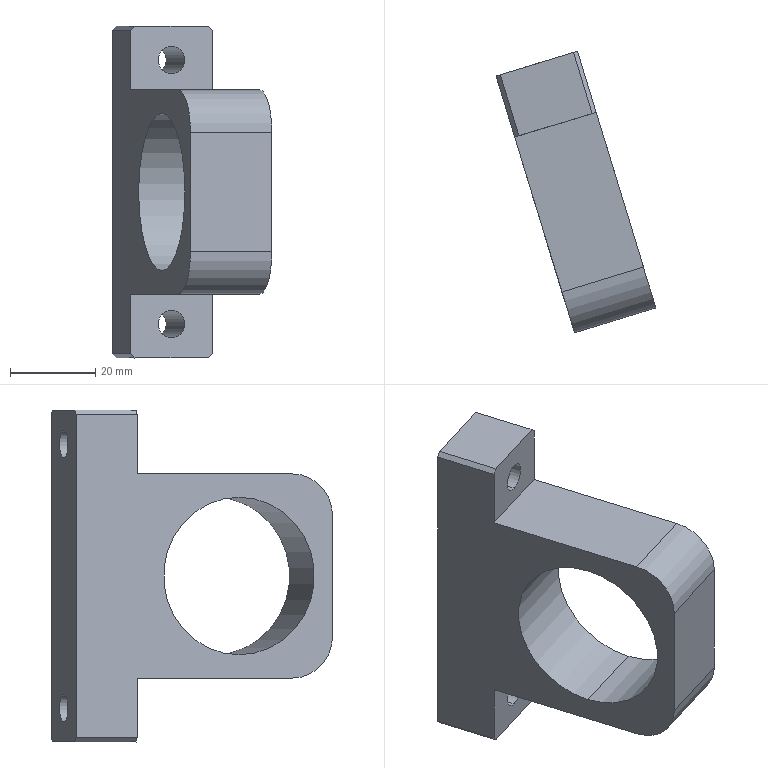Component | SolidWorks | V1ZHXTRotatingAxisMountingBaseSB1-1 | 1 solid | 22 faces | box 37.51 x 66.09 x 78 mm | volume 46092 mm3 | plane 14 | cylinder 8 | commonest cylinder face diameters 6.5 x4 37 x2 20 x2
build123d program:
from build123d import *

# Parameters (mm, degrees)
SKETCH1_W           = 20
SKETCH1_H           = 78
BOSS_EXTRUDE1_DEPTH = 63
SKETCH2_R           = 18.5
CUT_EXTRUDE1_DEPTH  = 77.746
SKETCH3_W           = 20
SKETCH3_H           = 15
CUT_EXTRUDE2_DEPTH  = 48
FILLET1_R           = 10
CHAMFER1_SIZE       = 1
SKETCH5_R           = 3.25
CUT_EXTRUDE3_DEPTH  = 66


with BuildPart() as part:
    # Sketch1 → Boss-Extrude1 (new body)
    with BuildSketch(Plane(origin=(0, 0, 0), x_dir=(1, 0, 0), z_dir=(0, 1, 0))):
        with Locations((10, 0)):
            Rectangle(SKETCH1_W, SKETCH1_H)
    extrude(amount=BOSS_EXTRUDE1_DEPTH)

    # Sketch2 → Cut-Extrude1 (cut, through all)
    with BuildSketch(Plane.ZY):
        with Locations((0, 40)):
            Circle(SKETCH2_R)
    extrude(amount=-CUT_EXTRUDE1_DEPTH, mode=Mode.SUBTRACT)

    # Sketch3 → Cut-Extrude2 (cut)
    with BuildSketch(Plane(origin=(0, 63, 0), x_dir=(1, 0, 0), z_dir=(0, 1, 0))):
        with Locations((10, -31.5)):
            Rectangle(SKETCH3_W, SKETCH3_H)
        with Locations((10, 31.5)):
            Rectangle(SKETCH3_W, SKETCH3_H)
    extrude(amount=-CUT_EXTRUDE2_DEPTH, mode=Mode.SUBTRACT)

    # Fillet1
    fillet1_edges = [part.edges().sort_by_distance(p)[0] for p in [
        (10, 63, 24),
        (10, 63, -24),
    ]]
    fillet(fillet1_edges, radius=FILLET1_R)

    # Chamfer1
    chamfer1_edges = [part.edges().sort_by_distance(p)[0] for p in [
        (20, 7.5, 39),
        (0, 7.5, 39),
        (0, 7.5, -39),
        (20, 7.5, -39),
    ]]
    chamfer(chamfer1_edges, length=CHAMFER1_SIZE)

    # Sketch5 → Cut-Extrude3 (cut, through all)
    with BuildSketch(Plane(origin=(0, 15, 0), x_dir=(1, 0, 0), z_dir=(0, 1, 0))):
        with Locations(Location((10, 31, 0), (0, 0, 270))):
            Circle(SKETCH5_R)
        with Locations(Location((10, -31, 0), (0, 0, 270))):
            Circle(SKETCH5_R)
    extrude(amount=-CUT_EXTRUDE3_DEPTH, mode=Mode.SUBTRACT)


solid = part.part

# Placed as in the assembly
solid = solid.moved(Location((215.737, -178.575, 375.239), (0, 0, -163.032)))
STEP:
#1=COLOUR_RGB('',0.7922,0.8196,0.9333);
#2=FILL_AREA_STYLE_COLOUR('',#1);
#3=FILL_AREA_STYLE('',(#2));
#4=SURFACE_STYLE_FILL_AREA(#3);
#5=SURFACE_SIDE_STYLE('',(#4));
#6=SURFACE_STYLE_USAGE(.BOTH.,#5);
#7=PRESENTATION_STYLE_ASSIGNMENT((#6));
#8=CARTESIAN_POINT('',(8.117,-7.145,15.866));
#9=VERTEX_POINT('',#8);
#10=CARTESIAN_POINT('',(8.117,-7.145,16.122));
#11=VERTEX_POINT('',#10);
#12=CARTESIAN_POINT('',(8.117,-7.145,15.994));
#13=DIRECTION('',(0.2918,-0.9565,-0.));
#14=DIRECTION('',(0.,-0.,1.));
#15=AXIS2_PLACEMENT_3D('',#12,#13,#14);
#16=CIRCLE('',#15,0.128);
#17=EDGE_CURVE('',#9,#11,#16,.T.);
#18=ORIENTED_EDGE('',*,*,#17,.F.);
#19=CARTESIAN_POINT('',(8.289,-7.71,15.866));
#20=VERTEX_POINT('',#19);
#21=CARTESIAN_POINT('',(8.117,-7.145,15.866));
#22=DIRECTION('',(0.2918,-0.9565,-0.));
#23=VECTOR('',#22,39.37);
#24=LINE('',#21,#23);
#25=EDGE_CURVE('',#9,#20,#24,.T.);
#26=ORIENTED_EDGE('',*,*,#25,.T.);
#27=CARTESIAN_POINT('',(8.289,-7.71,16.122));
#28=VERTEX_POINT('',#27);
#29=CARTESIAN_POINT('',(8.289,-7.71,15.994));
#30=DIRECTION('',(0.2918,-0.9565,-0.));
#31=DIRECTION('',(0.,-0.,1.));
#32=AXIS2_PLACEMENT_3D('',#29,#30,#31);
#33=CIRCLE('',#32,0.128);
#34=EDGE_CURVE('',#20,#28,#33,.T.);
#35=ORIENTED_EDGE('',*,*,#34,.T.);
#36=CARTESIAN_POINT('',(8.117,-7.145,16.122));
#37=DIRECTION('',(0.2918,-0.9565,-0.));
#38=VECTOR('',#37,39.37);
#39=LINE('',#36,#38);
#40=EDGE_CURVE('',#11,#28,#39,.T.);
#41=ORIENTED_EDGE('',*,*,#40,.F.);
#42=EDGE_LOOP('',(#18,#26,#35,#41));
#43=FACE_OUTER_BOUND('',#42,.T.);
#44=CARTESIAN_POINT('',(8.117,-7.145,15.994));
#45=DIRECTION('',(0.2918,-0.9565,-0.));
#46=DIRECTION('',(0.,-0.,1.));
#47=AXIS2_PLACEMENT_3D('',#44,#45,#46);
#48=CYLINDRICAL_SURFACE('',#47,0.128);
#49=ADVANCED_FACE('',(#43),#48,.F.);
#50=CARTESIAN_POINT('',(8.117,-7.145,13.425));
#51=VERTEX_POINT('',#50);
#52=CARTESIAN_POINT('',(8.117,-7.145,13.681));
#53=VERTEX_POINT('',#52);
#54=CARTESIAN_POINT('',(8.117,-7.145,13.553));
#55=DIRECTION('',(0.2918,-0.9565,-0.));
#56=DIRECTION('',(0.,-0.,1.));
#57=AXIS2_PLACEMENT_3D('',#54,#55,#56);
#58=CIRCLE('',#57,0.128);
#59=EDGE_CURVE('',#51,#53,#58,.T.);
#60=ORIENTED_EDGE('',*,*,#59,.F.);
#61=CARTESIAN_POINT('',(8.289,-7.71,13.425));
#62=VERTEX_POINT('',#61);
#63=CARTESIAN_POINT('',(8.117,-7.145,13.425));
#64=DIRECTION('',(0.2918,-0.9565,-0.));
#65=VECTOR('',#64,39.37);
#66=LINE('',#63,#65);
#67=EDGE_CURVE('',#51,#62,#66,.T.);
#68=ORIENTED_EDGE('',*,*,#67,.T.);
#69=CARTESIAN_POINT('',(8.289,-7.71,13.681));
#70=VERTEX_POINT('',#69);
#71=CARTESIAN_POINT('',(8.289,-7.71,13.553));
#72=DIRECTION('',(0.2918,-0.9565,-0.));
#73=DIRECTION('',(0.,-0.,1.));
#74=AXIS2_PLACEMENT_3D('',#71,#72,#73);
#75=CIRCLE('',#74,0.128);
#76=EDGE_CURVE('',#62,#70,#75,.T.);
#77=ORIENTED_EDGE('',*,*,#76,.T.);
#78=CARTESIAN_POINT('',(8.117,-7.145,13.681));
#79=DIRECTION('',(0.2918,-0.9565,-0.));
#80=VECTOR('',#79,39.37);
#81=LINE('',#78,#80);
#82=EDGE_CURVE('',#53,#70,#81,.T.);
#83=ORIENTED_EDGE('',*,*,#82,.F.);
#84=EDGE_LOOP('',(#60,#68,#77,#83));
#85=FACE_OUTER_BOUND('',#84,.T.);
#86=CARTESIAN_POINT('',(8.117,-7.145,13.553));
#87=DIRECTION('',(0.2918,-0.9565,-0.));
#88=DIRECTION('',(0.,-0.,1.));
#89=AXIS2_PLACEMENT_3D('',#86,#87,#88);
#90=CYLINDRICAL_SURFACE('',#89,0.128);
#91=ADVANCED_FACE('',(#85),#90,.F.);
#92=CARTESIAN_POINT('',(8.2,-8.767,14.045));
#93=VERTEX_POINT('',#92);
#94=CARTESIAN_POINT('',(8.2,-8.767,15.502));
#95=VERTEX_POINT('',#94);
#96=CARTESIAN_POINT('',(8.2,-8.767,14.773));
#97=DIRECTION('',(0.9565,0.2918,0.));
#98=DIRECTION('',(-0.,-0.,1.));
#99=AXIS2_PLACEMENT_3D('',#96,#97,#98);
#100=CIRCLE('',#99,0.7283);
#101=EDGE_CURVE('',#93,#95,#100,.T.);
#102=ORIENTED_EDGE('',*,*,#101,.F.);
#103=CARTESIAN_POINT('',(8.953,-8.537,14.045));
#104=VERTEX_POINT('',#103);
#105=CARTESIAN_POINT('',(8.2,-8.767,14.045));
#106=DIRECTION('',(0.9565,0.2918,0.));
#107=VECTOR('',#106,39.37);
#108=LINE('',#105,#107);
#109=EDGE_CURVE('',#93,#104,#108,.T.);
#110=ORIENTED_EDGE('',*,*,#109,.T.);
#111=CARTESIAN_POINT('',(8.953,-8.537,15.502));
#112=VERTEX_POINT('',#111);
#113=CARTESIAN_POINT('',(8.953,-8.537,14.773));
#114=DIRECTION('',(0.9565,0.2918,0.));
#115=DIRECTION('',(-0.,-0.,1.));
#116=AXIS2_PLACEMENT_3D('',#113,#114,#115);
#117=CIRCLE('',#116,0.7283);
#118=EDGE_CURVE('',#104,#112,#117,.T.);
#119=ORIENTED_EDGE('',*,*,#118,.T.);
#120=CARTESIAN_POINT('',(8.2,-8.767,15.502));
#121=DIRECTION('',(0.9565,0.2918,0.));
#122=VECTOR('',#121,39.37);
#123=LINE('',#120,#122);
#124=EDGE_CURVE('',#95,#112,#123,.T.);
#125=ORIENTED_EDGE('',*,*,#124,.F.);
#126=EDGE_LOOP('',(#102,#110,#119,#125));
#127=FACE_OUTER_BOUND('',#126,.T.);
#128=CARTESIAN_POINT('',(8.2,-8.767,14.773));
#129=DIRECTION('',(0.9565,0.2918,0.));
#130=DIRECTION('',(-0.,-0.,1.));
#131=AXIS2_PLACEMENT_3D('',#128,#129,#130);
#132=CYLINDRICAL_SURFACE('',#131,0.7283);
#133=ADVANCED_FACE('',(#127),#132,.F.);
#134=CARTESIAN_POINT('',(7.95,-7.814,13.238));
#135=VERTEX_POINT('',#134);
#136=CARTESIAN_POINT('',(8.628,-7.607,13.238));
#137=VERTEX_POINT('',#136);
#138=CARTESIAN_POINT('',(8.666,-7.595,13.238));
#139=DIRECTION('',(0.9565,0.2918,0.));
#140=VECTOR('',#139,39.37);
#141=LINE('',#138,#140);
#142=EDGE_CURVE('',#135,#137,#141,.T.);
#143=ORIENTED_EDGE('',*,*,#142,.F.);
#144=CARTESIAN_POINT('',(7.778,-7.249,13.238));
#145=VERTEX_POINT('',#144);
#146=CARTESIAN_POINT('',(8.502,-9.621,13.238));
#147=DIRECTION('',(-0.2918,0.9565,0.));
#148=VECTOR('',#147,39.37);
#149=LINE('',#146,#148);
#150=EDGE_CURVE('',#135,#145,#149,.T.);
#151=ORIENTED_EDGE('',*,*,#150,.T.);
#152=CARTESIAN_POINT('',(8.456,-7.042,13.238));
#153=VERTEX_POINT('',#152);
#154=CARTESIAN_POINT('',(8.494,-7.031,13.238));
#155=DIRECTION('',(0.9565,0.2918,0.));
#156=VECTOR('',#155,39.37);
#157=LINE('',#154,#156);
#158=EDGE_CURVE('',#145,#153,#157,.T.);
#159=ORIENTED_EDGE('',*,*,#158,.T.);
#160=CARTESIAN_POINT('',(9.18,-9.414,13.238));
#161=DIRECTION('',(0.2918,-0.9565,-0.));
#162=VECTOR('',#161,39.37);
#163=LINE('',#160,#162);
#164=EDGE_CURVE('',#153,#137,#163,.T.);
#165=ORIENTED_EDGE('',*,*,#164,.T.);
#166=EDGE_LOOP('',(#143,#151,#159,#165));
#167=FACE_OUTER_BOUND('',#166,.T.);
#168=CARTESIAN_POINT('',(9.217,-9.403,13.238));
#169=DIRECTION('',(-0.,-0.,1.));
#170=DIRECTION('',(-0.9565,-0.2918,-0.));
#171=AXIS2_PLACEMENT_3D('',#168,#169,#170);
#172=PLANE('',#171);
#173=ADVANCED_FACE('',(#167),#172,.F.);
#174=CARTESIAN_POINT('',(8.953,-8.537,14.773));
#175=DIRECTION('',(0.9565,0.2918,0.));
#176=DIRECTION('',(-0.,-0.,1.));
#177=AXIS2_PLACEMENT_3D('',#174,#175,#176);
#178=CIRCLE('',#177,0.7283);
#179=EDGE_CURVE('',#112,#104,#178,.T.);
#180=ORIENTED_EDGE('',*,*,#179,.F.);
#181=ORIENTED_EDGE('',*,*,#118,.F.);
#182=EDGE_LOOP('',(#180,#181));
#183=FACE_BOUND('',#182,.T.);
#184=CARTESIAN_POINT('',(8.494,-7.031,13.277));
#185=VERTEX_POINT('',#184);
#186=CARTESIAN_POINT('',(8.494,-7.031,16.269));
#187=VERTEX_POINT('',#186);
#188=CARTESIAN_POINT('',(8.494,-7.031,13.238));
#189=DIRECTION('',(-0.,-0.,1.));
#190=VECTOR('',#189,39.37);
#191=LINE('',#188,#190);
#192=EDGE_CURVE('',#185,#187,#191,.T.);
#193=ORIENTED_EDGE('',*,*,#192,.T.);
#194=CARTESIAN_POINT('',(8.666,-7.595,16.269));
#195=VERTEX_POINT('',#194);
#196=CARTESIAN_POINT('',(9.217,-9.403,16.269));
#197=DIRECTION('',(0.2918,-0.9565,-0.));
#198=VECTOR('',#197,39.37);
#199=LINE('',#196,#198);
#200=EDGE_CURVE('',#187,#195,#199,.T.);
#201=ORIENTED_EDGE('',*,*,#200,.T.);
#202=CARTESIAN_POINT('',(8.666,-7.595,15.718));
#203=VERTEX_POINT('',#202);
#204=CARTESIAN_POINT('',(8.666,-7.595,16.309));
#205=DIRECTION('',(-0.,-0.,1.));
#206=VECTOR('',#205,39.37);
#207=LINE('',#204,#206);
#208=EDGE_CURVE('',#203,#195,#207,.T.);
#209=ORIENTED_EDGE('',*,*,#208,.F.);
#210=CARTESIAN_POINT('',(9.103,-9.026,15.718));
#211=VERTEX_POINT('',#210);
#212=CARTESIAN_POINT('',(8.666,-7.595,15.718));
#213=DIRECTION('',(0.2918,-0.9565,-0.));
#214=VECTOR('',#213,39.37);
#215=LINE('',#212,#214);
#216=EDGE_CURVE('',#203,#211,#215,.T.);
#217=ORIENTED_EDGE('',*,*,#216,.T.);
#218=CARTESIAN_POINT('',(9.217,-9.403,15.324));
#219=VERTEX_POINT('',#218);
#220=CARTESIAN_POINT('',(9.103,-9.026,15.324));
#221=DIRECTION('',(0.9565,0.2918,0.));
#222=DIRECTION('',(0.,0.,-1.));
#223=AXIS2_PLACEMENT_3D('',#220,#221,#222);
#224=CIRCLE('',#223,0.3937);
#225=EDGE_CURVE('',#211,#219,#224,.T.);
#226=ORIENTED_EDGE('',*,*,#225,.T.);
#227=CARTESIAN_POINT('',(9.217,-9.403,14.222));
#228=VERTEX_POINT('',#227);
#229=CARTESIAN_POINT('',(9.217,-9.403,13.238));
#230=DIRECTION('',(-0.,-0.,1.));
#231=VECTOR('',#230,39.37);
#232=LINE('',#229,#231);
#233=EDGE_CURVE('',#228,#219,#232,.T.);
#234=ORIENTED_EDGE('',*,*,#233,.F.);
#235=CARTESIAN_POINT('',(9.103,-9.026,13.828));
#236=VERTEX_POINT('',#235);
#237=CARTESIAN_POINT('',(9.103,-9.026,14.222));
#238=DIRECTION('',(0.9565,0.2918,0.));
#239=DIRECTION('',(0.,0.,-1.));
#240=AXIS2_PLACEMENT_3D('',#237,#238,#239);
#241=CIRCLE('',#240,0.3937);
#242=EDGE_CURVE('',#228,#236,#241,.T.);
#243=ORIENTED_EDGE('',*,*,#242,.T.);
#244=CARTESIAN_POINT('',(8.666,-7.595,13.828));
#245=VERTEX_POINT('',#244);
#246=CARTESIAN_POINT('',(8.666,-7.595,13.828));
#247=DIRECTION('',(0.2918,-0.9565,-0.));
#248=VECTOR('',#247,39.37);
#249=LINE('',#246,#248);
#250=EDGE_CURVE('',#245,#236,#249,.T.);
#251=ORIENTED_EDGE('',*,*,#250,.F.);
#252=CARTESIAN_POINT('',(8.666,-7.595,13.277));
#253=VERTEX_POINT('',#252);
#254=CARTESIAN_POINT('',(8.666,-7.595,13.238));
#255=DIRECTION('',(-0.,-0.,1.));
#256=VECTOR('',#255,39.37);
#257=LINE('',#254,#256);
#258=EDGE_CURVE('',#253,#245,#257,.T.);
#259=ORIENTED_EDGE('',*,*,#258,.F.);
#260=CARTESIAN_POINT('',(9.217,-9.403,13.277));
#261=DIRECTION('',(-0.2918,0.9565,0.));
#262=VECTOR('',#261,39.37);
#263=LINE('',#260,#262);
#264=EDGE_CURVE('',#253,#185,#263,.T.);
#265=ORIENTED_EDGE('',*,*,#264,.T.);
#266=EDGE_LOOP('',(#193,#201,#209,#217,#226,#234,#243,#251,#259,#265));
#267=FACE_OUTER_BOUND('',#266,.T.);
#268=CARTESIAN_POINT('',(9.217,-9.403,13.238));
#269=DIRECTION('',(-0.9565,-0.2918,-0.));
#270=DIRECTION('',(0.,0.,-1.));
#271=AXIS2_PLACEMENT_3D('',#268,#269,#270);
#272=PLANE('',#271);
#273=ADVANCED_FACE('',(#183,#267),#272,.F.);
#274=CARTESIAN_POINT('',(8.456,-7.042,16.309));
#275=VERTEX_POINT('',#274);
#276=CARTESIAN_POINT('',(7.778,-7.249,16.309));
#277=VERTEX_POINT('',#276);
#278=CARTESIAN_POINT('',(8.494,-7.031,16.309));
#279=DIRECTION('',(-0.9565,-0.2918,-0.));
#280=VECTOR('',#279,39.37);
#281=LINE('',#278,#280);
#282=EDGE_CURVE('',#275,#277,#281,.T.);
#283=ORIENTED_EDGE('',*,*,#282,.T.);
#284=CARTESIAN_POINT('',(7.95,-7.814,16.309));
#285=VERTEX_POINT('',#284);
#286=CARTESIAN_POINT('',(8.502,-9.621,16.309));
#287=DIRECTION('',(0.2918,-0.9565,-0.));
#288=VECTOR('',#287,39.37);
#289=LINE('',#286,#288);
#290=EDGE_CURVE('',#277,#285,#289,.T.);
#291=ORIENTED_EDGE('',*,*,#290,.T.);
#292=CARTESIAN_POINT('',(8.628,-7.607,16.309));
#293=VERTEX_POINT('',#292);
#294=CARTESIAN_POINT('',(8.666,-7.595,16.309));
#295=DIRECTION('',(-0.9565,-0.2918,-0.));
#296=VECTOR('',#295,39.37);
#297=LINE('',#294,#296);
#298=EDGE_CURVE('',#293,#285,#297,.T.);
#299=ORIENTED_EDGE('',*,*,#298,.F.);
#300=CARTESIAN_POINT('',(9.18,-9.414,16.309));
#301=DIRECTION('',(-0.2918,0.9565,0.));
#302=VECTOR('',#301,39.37);
#303=LINE('',#300,#302);
#304=EDGE_CURVE('',#293,#275,#303,.T.);
#305=ORIENTED_EDGE('',*,*,#304,.T.);
#306=EDGE_LOOP('',(#283,#291,#299,#305));
#307=FACE_OUTER_BOUND('',#306,.T.);
#308=CARTESIAN_POINT('',(9.217,-9.403,16.309));
#309=DIRECTION('',(0.,0.,-1.));
#310=DIRECTION('',(0.9565,0.2918,0.));
#311=AXIS2_PLACEMENT_3D('',#308,#309,#310);
#312=PLANE('',#311);
#313=ADVANCED_FACE('',(#307),#312,.F.);
#314=CARTESIAN_POINT('',(8.2,-8.767,14.773));
#315=DIRECTION('',(0.9565,0.2918,0.));
#316=DIRECTION('',(-0.,-0.,1.));
#317=AXIS2_PLACEMENT_3D('',#314,#315,#316);
#318=CIRCLE('',#317,0.7283);
#319=EDGE_CURVE('',#95,#93,#318,.T.);
#320=ORIENTED_EDGE('',*,*,#319,.T.);
#321=ORIENTED_EDGE('',*,*,#101,.T.);
#322=EDGE_LOOP('',(#320,#321));
#323=FACE_BOUND('',#322,.T.);
#324=CARTESIAN_POINT('',(7.74,-7.26,16.269));
#325=VERTEX_POINT('',#324);
#326=CARTESIAN_POINT('',(7.74,-7.26,13.277));
#327=VERTEX_POINT('',#326);
#328=CARTESIAN_POINT('',(7.74,-7.26,13.238));
#329=DIRECTION('',(0.,0.,-1.));
#330=VECTOR('',#329,39.37);
#331=LINE('',#328,#330);
#332=EDGE_CURVE('',#325,#327,#331,.T.);
#333=ORIENTED_EDGE('',*,*,#332,.T.);
#334=CARTESIAN_POINT('',(7.913,-7.825,13.277));
#335=VERTEX_POINT('',#334);
#336=CARTESIAN_POINT('',(8.464,-9.633,13.277));
#337=DIRECTION('',(0.2918,-0.9565,-0.));
#338=VECTOR('',#337,39.37);
#339=LINE('',#336,#338);
#340=EDGE_CURVE('',#327,#335,#339,.T.);
#341=ORIENTED_EDGE('',*,*,#340,.T.);
#342=CARTESIAN_POINT('',(7.913,-7.825,13.828));
#343=VERTEX_POINT('',#342);
#344=CARTESIAN_POINT('',(7.913,-7.825,13.238));
#345=DIRECTION('',(0.,0.,-1.));
#346=VECTOR('',#345,39.37);
#347=LINE('',#344,#346);
#348=EDGE_CURVE('',#343,#335,#347,.T.);
#349=ORIENTED_EDGE('',*,*,#348,.F.);
#350=CARTESIAN_POINT('',(8.349,-9.256,13.828));
#351=VERTEX_POINT('',#350);
#352=CARTESIAN_POINT('',(7.913,-7.825,13.828));
#353=DIRECTION('',(0.2918,-0.9565,-0.));
#354=VECTOR('',#353,39.37);
#355=LINE('',#352,#354);
#356=EDGE_CURVE('',#343,#351,#355,.T.);
#357=ORIENTED_EDGE('',*,*,#356,.T.);
#358=CARTESIAN_POINT('',(8.464,-9.633,14.222));
#359=VERTEX_POINT('',#358);
#360=CARTESIAN_POINT('',(8.349,-9.256,14.222));
#361=DIRECTION('',(-0.9565,-0.2918,-0.));
#362=DIRECTION('',(-0.,-0.,1.));
#363=AXIS2_PLACEMENT_3D('',#360,#361,#362);
#364=CIRCLE('',#363,0.3937);
#365=EDGE_CURVE('',#351,#359,#364,.T.);
#366=ORIENTED_EDGE('',*,*,#365,.T.);
#367=CARTESIAN_POINT('',(8.464,-9.633,15.324));
#368=VERTEX_POINT('',#367);
#369=CARTESIAN_POINT('',(8.464,-9.633,13.238));
#370=DIRECTION('',(0.,0.,-1.));
#371=VECTOR('',#370,39.37);
#372=LINE('',#369,#371);
#373=EDGE_CURVE('',#368,#359,#372,.T.);
#374=ORIENTED_EDGE('',*,*,#373,.F.);
#375=CARTESIAN_POINT('',(8.349,-9.256,15.718));
#376=VERTEX_POINT('',#375);
#377=CARTESIAN_POINT('',(8.349,-9.256,15.324));
#378=DIRECTION('',(-0.9565,-0.2918,-0.));
#379=DIRECTION('',(-0.,-0.,1.));
#380=AXIS2_PLACEMENT_3D('',#377,#378,#379);
#381=CIRCLE('',#380,0.3937);
#382=EDGE_CURVE('',#368,#376,#381,.T.);
#383=ORIENTED_EDGE('',*,*,#382,.T.);
#384=CARTESIAN_POINT('',(7.913,-7.825,15.718));
#385=VERTEX_POINT('',#384);
#386=CARTESIAN_POINT('',(7.913,-7.825,15.718));
#387=DIRECTION('',(0.2918,-0.9565,-0.));
#388=VECTOR('',#387,39.37);
#389=LINE('',#386,#388);
#390=EDGE_CURVE('',#385,#376,#389,.T.);
#391=ORIENTED_EDGE('',*,*,#390,.F.);
#392=CARTESIAN_POINT('',(7.913,-7.825,16.269));
#393=VERTEX_POINT('',#392);
#394=CARTESIAN_POINT('',(7.913,-7.825,16.309));
#395=DIRECTION('',(0.,0.,-1.));
#396=VECTOR('',#395,39.37);
#397=LINE('',#394,#396);
#398=EDGE_CURVE('',#393,#385,#397,.T.);
#399=ORIENTED_EDGE('',*,*,#398,.F.);
#400=CARTESIAN_POINT('',(8.464,-9.633,16.269));
#401=DIRECTION('',(-0.2918,0.9565,0.));
#402=VECTOR('',#401,39.37);
#403=LINE('',#400,#402);
#404=EDGE_CURVE('',#393,#325,#403,.T.);
#405=ORIENTED_EDGE('',*,*,#404,.T.);
#406=EDGE_LOOP('',(#333,#341,#349,#357,#366,#374,#383,#391,#399,#405));
#407=FACE_OUTER_BOUND('',#406,.T.);
#408=CARTESIAN_POINT('',(8.464,-9.633,13.238));
#409=DIRECTION('',(0.9565,0.2918,0.));
#410=DIRECTION('',(-0.,-0.,1.));
#411=AXIS2_PLACEMENT_3D('',#408,#409,#410);
#412=PLANE('',#411);
#413=ADVANCED_FACE('',(#323,#407),#412,.F.);
#414=ORIENTED_EDGE('',*,*,#233,.T.);
#415=CARTESIAN_POINT('',(8.464,-9.633,15.324));
#416=DIRECTION('',(-0.9565,-0.2918,-0.));
#417=VECTOR('',#416,39.37);
#418=LINE('',#415,#417);
#419=EDGE_CURVE('',#219,#368,#418,.T.);
#420=ORIENTED_EDGE('',*,*,#419,.T.);
#421=ORIENTED_EDGE('',*,*,#373,.T.);
#422=CARTESIAN_POINT('',(9.217,-9.403,14.222));
#423=DIRECTION('',(0.9565,0.2918,0.));
#424=VECTOR('',#423,39.37);
#425=LINE('',#422,#424);
#426=EDGE_CURVE('',#359,#228,#425,.T.);
#427=ORIENTED_EDGE('',*,*,#426,.T.);
#428=EDGE_LOOP('',(#414,#420,#421,#427));
#429=FACE_OUTER_BOUND('',#428,.T.);
#430=CARTESIAN_POINT('',(9.217,-9.403,14.773));
#431=DIRECTION('',(0.2918,-0.9565,-0.));
#432=DIRECTION('',(-0.,-0.,1.));
#433=AXIS2_PLACEMENT_3D('',#430,#431,#432);
#434=PLANE('',#433);
#435=ADVANCED_FACE('',(#429),#434,.T.);
#436=CARTESIAN_POINT('',(8.117,-7.145,15.994));
#437=DIRECTION('',(0.2918,-0.9565,-0.));
#438=DIRECTION('',(0.,-0.,1.));
#439=AXIS2_PLACEMENT_3D('',#436,#437,#438);
#440=CIRCLE('',#439,0.128);
#441=EDGE_CURVE('',#11,#9,#440,.T.);
#442=ORIENTED_EDGE('',*,*,#441,.T.);
#443=ORIENTED_EDGE('',*,*,#17,.T.);
#444=EDGE_LOOP('',(#442,#443));
#445=FACE_BOUND('',#444,.T.);
#446=CARTESIAN_POINT('',(8.117,-7.145,13.553));
#447=DIRECTION('',(0.2918,-0.9565,-0.));
#448=DIRECTION('',(0.,-0.,1.));
#449=AXIS2_PLACEMENT_3D('',#446,#447,#448);
#450=CIRCLE('',#449,0.128);
#451=EDGE_CURVE('',#53,#51,#450,.T.);
#452=ORIENTED_EDGE('',*,*,#451,.T.);
#453=ORIENTED_EDGE('',*,*,#59,.T.);
#454=EDGE_LOOP('',(#452,#453));
#455=FACE_BOUND('',#454,.T.);
#456=ORIENTED_EDGE('',*,*,#158,.F.);
#457=CARTESIAN_POINT('',(7.778,-7.249,13.238));
#458=DIRECTION('',(-0.6763,-0.2064,0.7071));
#459=VECTOR('',#458,39.37);
#460=LINE('',#457,#459);
#461=EDGE_CURVE('',#145,#327,#460,.T.);
#462=ORIENTED_EDGE('',*,*,#461,.T.);
#463=ORIENTED_EDGE('',*,*,#332,.F.);
#464=CARTESIAN_POINT('',(7.74,-7.26,16.269));
#465=DIRECTION('',(0.6763,0.2064,0.7071));
#466=VECTOR('',#465,39.37);
#467=LINE('',#464,#466);
#468=EDGE_CURVE('',#325,#277,#467,.T.);
#469=ORIENTED_EDGE('',*,*,#468,.T.);
#470=ORIENTED_EDGE('',*,*,#282,.F.);
#471=CARTESIAN_POINT('',(8.456,-7.042,16.309));
#472=DIRECTION('',(0.6763,0.2064,-0.7071));
#473=VECTOR('',#472,39.37);
#474=LINE('',#471,#473);
#475=EDGE_CURVE('',#275,#187,#474,.T.);
#476=ORIENTED_EDGE('',*,*,#475,.T.);
#477=ORIENTED_EDGE('',*,*,#192,.F.);
#478=CARTESIAN_POINT('',(8.494,-7.031,13.277));
#479=DIRECTION('',(-0.6763,-0.2064,-0.7071));
#480=VECTOR('',#479,39.37);
#481=LINE('',#478,#480);
#482=EDGE_CURVE('',#185,#153,#481,.T.);
#483=ORIENTED_EDGE('',*,*,#482,.T.);
#484=EDGE_LOOP('',(#456,#462,#463,#469,#470,#476,#477,#483));
#485=FACE_OUTER_BOUND('',#484,.T.);
#486=CARTESIAN_POINT('',(8.494,-7.031,14.773));
#487=DIRECTION('',(0.2918,-0.9565,-0.));
#488=DIRECTION('',(-0.,-0.,1.));
#489=AXIS2_PLACEMENT_3D('',#486,#487,#488);
#490=PLANE('',#489);
#491=ADVANCED_FACE('',(#445,#455,#485),#490,.F.);
#492=ORIENTED_EDGE('',*,*,#109,.F.);
#493=ORIENTED_EDGE('',*,*,#319,.F.);
#494=ORIENTED_EDGE('',*,*,#124,.T.);
#495=ORIENTED_EDGE('',*,*,#179,.T.);
#496=EDGE_LOOP('',(#492,#493,#494,#495));
#497=FACE_OUTER_BOUND('',#496,.T.);
#498=CARTESIAN_POINT('',(8.2,-8.767,14.773));
#499=DIRECTION('',(0.9565,0.2918,0.));
#500=DIRECTION('',(-0.,-0.,1.));
#501=AXIS2_PLACEMENT_3D('',#498,#499,#500);
#502=CYLINDRICAL_SURFACE('',#501,0.7283);
#503=ADVANCED_FACE('',(#497),#502,.F.);
#504=ORIENTED_EDGE('',*,*,#390,.T.);
#505=CARTESIAN_POINT('',(9.103,-9.026,15.718));
#506=DIRECTION('',(0.9565,0.2918,0.));
#507=VECTOR('',#506,39.37);
#508=LINE('',#505,#507);
#509=EDGE_CURVE('',#376,#211,#508,.T.);
#510=ORIENTED_EDGE('',*,*,#509,.T.);
#511=ORIENTED_EDGE('',*,*,#216,.F.);
#512=CARTESIAN_POINT('',(8.666,-7.595,15.718));
#513=DIRECTION('',(0.9565,0.2918,0.));
#514=VECTOR('',#513,39.37);
#515=LINE('',#512,#514);
#516=EDGE_CURVE('',#385,#203,#515,.T.);
#517=ORIENTED_EDGE('',*,*,#516,.F.);
#518=EDGE_LOOP('',(#504,#510,#511,#517));
#519=FACE_OUTER_BOUND('',#518,.T.);
#520=CARTESIAN_POINT('',(8.666,-7.595,15.718));
#521=DIRECTION('',(0.,0.,-1.));
#522=DIRECTION('',(0.9565,0.2918,0.));
#523=AXIS2_PLACEMENT_3D('',#520,#521,#522);
#524=PLANE('',#523);
#525=ADVANCED_FACE('',(#519),#524,.F.);
#526=CARTESIAN_POINT('',(8.289,-7.71,15.994));
#527=DIRECTION('',(0.2918,-0.9565,-0.));
#528=DIRECTION('',(0.,-0.,1.));
#529=AXIS2_PLACEMENT_3D('',#526,#527,#528);
#530=CIRCLE('',#529,0.128);
#531=EDGE_CURVE('',#28,#20,#530,.T.);
#532=ORIENTED_EDGE('',*,*,#531,.F.);
#533=ORIENTED_EDGE('',*,*,#34,.F.);
#534=EDGE_LOOP('',(#532,#533));
#535=FACE_BOUND('',#534,.T.);
#536=ORIENTED_EDGE('',*,*,#298,.T.);
#537=CARTESIAN_POINT('',(7.913,-7.825,16.269));
#538=DIRECTION('',(-0.6763,-0.2064,-0.7071));
#539=VECTOR('',#538,39.37);
#540=LINE('',#537,#539);
#541=EDGE_CURVE('',#285,#393,#540,.T.);
#542=ORIENTED_EDGE('',*,*,#541,.T.);
#543=ORIENTED_EDGE('',*,*,#398,.T.);
#544=ORIENTED_EDGE('',*,*,#516,.T.);
#545=ORIENTED_EDGE('',*,*,#208,.T.);
#546=CARTESIAN_POINT('',(8.628,-7.607,16.309));
#547=DIRECTION('',(-0.6763,-0.2064,0.7071));
#548=VECTOR('',#547,39.37);
#549=LINE('',#546,#548);
#550=EDGE_CURVE('',#195,#293,#549,.T.);
#551=ORIENTED_EDGE('',*,*,#550,.T.);
#552=EDGE_LOOP('',(#536,#542,#543,#544,#545,#551));
#553=FACE_OUTER_BOUND('',#552,.T.);
#554=CARTESIAN_POINT('',(8.666,-7.595,14.773));
#555=DIRECTION('',(-0.2918,0.9565,0.));
#556=DIRECTION('',(0.,0.,-1.));
#557=AXIS2_PLACEMENT_3D('',#554,#555,#556);
#558=PLANE('',#557);
#559=ADVANCED_FACE('',(#535,#553),#558,.F.);
#560=ORIENTED_EDGE('',*,*,#250,.T.);
#561=CARTESIAN_POINT('',(8.349,-9.256,13.828));
#562=DIRECTION('',(-0.9565,-0.2918,-0.));
#563=VECTOR('',#562,39.37);
#564=LINE('',#561,#563);
#565=EDGE_CURVE('',#236,#351,#564,.T.);
#566=ORIENTED_EDGE('',*,*,#565,.T.);
#567=ORIENTED_EDGE('',*,*,#356,.F.);
#568=CARTESIAN_POINT('',(8.666,-7.595,13.828));
#569=DIRECTION('',(-0.9565,-0.2918,-0.));
#570=VECTOR('',#569,39.37);
#571=LINE('',#568,#570);
#572=EDGE_CURVE('',#245,#343,#571,.T.);
#573=ORIENTED_EDGE('',*,*,#572,.F.);
#574=EDGE_LOOP('',(#560,#566,#567,#573));
#575=FACE_OUTER_BOUND('',#574,.T.);
#576=CARTESIAN_POINT('',(8.666,-7.595,13.828));
#577=DIRECTION('',(-0.,-0.,1.));
#578=DIRECTION('',(-0.9565,-0.2918,-0.));
#579=AXIS2_PLACEMENT_3D('',#576,#577,#578);
#580=PLANE('',#579);
#581=ADVANCED_FACE('',(#575),#580,.F.);
#582=CARTESIAN_POINT('',(8.289,-7.71,13.553));
#583=DIRECTION('',(0.2918,-0.9565,-0.));
#584=DIRECTION('',(0.,-0.,1.));
#585=AXIS2_PLACEMENT_3D('',#582,#583,#584);
#586=CIRCLE('',#585,0.128);
#587=EDGE_CURVE('',#70,#62,#586,.T.);
#588=ORIENTED_EDGE('',*,*,#587,.F.);
#589=ORIENTED_EDGE('',*,*,#76,.F.);
#590=EDGE_LOOP('',(#588,#589));
#591=FACE_BOUND('',#590,.T.);
#592=ORIENTED_EDGE('',*,*,#348,.T.);
#593=CARTESIAN_POINT('',(7.574,-7.929,13.631));
#594=DIRECTION('',(0.6763,0.2064,-0.7071));
#595=VECTOR('',#594,39.37);
#596=LINE('',#593,#595);
#597=EDGE_CURVE('',#335,#135,#596,.T.);
#598=ORIENTED_EDGE('',*,*,#597,.T.);
#599=ORIENTED_EDGE('',*,*,#142,.T.);
#600=CARTESIAN_POINT('',(9.381,-7.377,14.025));
#601=DIRECTION('',(0.6763,0.2064,0.7071));
#602=VECTOR('',#601,39.37);
#603=LINE('',#600,#602);
#604=EDGE_CURVE('',#137,#253,#603,.T.);
#605=ORIENTED_EDGE('',*,*,#604,.T.);
#606=ORIENTED_EDGE('',*,*,#258,.T.);
#607=ORIENTED_EDGE('',*,*,#572,.T.);
#608=EDGE_LOOP('',(#592,#598,#599,#605,#606,#607));
#609=FACE_OUTER_BOUND('',#608,.T.);
#610=CARTESIAN_POINT('',(8.666,-7.595,14.773));
#611=DIRECTION('',(0.2918,-0.9565,-0.));
#612=DIRECTION('',(-0.,-0.,1.));
#613=AXIS2_PLACEMENT_3D('',#610,#611,#612);
#614=PLANE('',#613);
#615=ADVANCED_FACE('',(#591,#609),#614,.T.);
#616=ORIENTED_EDGE('',*,*,#382,.F.);
#617=ORIENTED_EDGE('',*,*,#419,.F.);
#618=ORIENTED_EDGE('',*,*,#225,.F.);
#619=ORIENTED_EDGE('',*,*,#509,.F.);
#620=EDGE_LOOP('',(#616,#617,#618,#619));
#621=FACE_OUTER_BOUND('',#620,.T.);
#622=CARTESIAN_POINT('',(9.103,-9.026,15.324));
#623=DIRECTION('',(-0.9565,-0.2918,-0.));
#624=DIRECTION('',(0.,0.,-1.));
#625=AXIS2_PLACEMENT_3D('',#622,#623,#624);
#626=CYLINDRICAL_SURFACE('',#625,0.3937);
#627=ADVANCED_FACE('',(#621),#626,.T.);
#628=ORIENTED_EDGE('',*,*,#242,.F.);
#629=ORIENTED_EDGE('',*,*,#426,.F.);
#630=ORIENTED_EDGE('',*,*,#365,.F.);
#631=ORIENTED_EDGE('',*,*,#565,.F.);
#632=EDGE_LOOP('',(#628,#629,#630,#631));
#633=FACE_OUTER_BOUND('',#632,.T.);
#634=CARTESIAN_POINT('',(9.103,-9.026,14.222));
#635=DIRECTION('',(0.9565,0.2918,0.));
#636=DIRECTION('',(-0.,-0.,1.));
#637=AXIS2_PLACEMENT_3D('',#634,#635,#636);
#638=CYLINDRICAL_SURFACE('',#637,0.3937);
#639=ADVANCED_FACE('',(#633),#638,.T.);
#640=ORIENTED_EDGE('',*,*,#597,.F.);
#641=ORIENTED_EDGE('',*,*,#340,.F.);
#642=ORIENTED_EDGE('',*,*,#461,.F.);
#643=ORIENTED_EDGE('',*,*,#150,.F.);
#644=EDGE_LOOP('',(#640,#641,#642,#643));
#645=FACE_OUTER_BOUND('',#644,.T.);
#646=CARTESIAN_POINT('',(8.502,-9.621,13.238));
#647=DIRECTION('',(0.6763,0.2064,0.7071));
#648=DIRECTION('',(-0.2918,0.9565,0.));
#649=AXIS2_PLACEMENT_3D('',#646,#647,#648);
#650=PLANE('',#649);
#651=ADVANCED_FACE('',(#645),#650,.F.);
#652=ORIENTED_EDGE('',*,*,#541,.F.);
#653=ORIENTED_EDGE('',*,*,#290,.F.);
#654=ORIENTED_EDGE('',*,*,#468,.F.);
#655=ORIENTED_EDGE('',*,*,#404,.F.);
#656=EDGE_LOOP('',(#652,#653,#654,#655));
#657=FACE_OUTER_BOUND('',#656,.T.);
#658=CARTESIAN_POINT('',(8.464,-9.633,16.269));
#659=DIRECTION('',(0.6763,0.2064,-0.7071));
#660=DIRECTION('',(-0.2918,0.9565,0.));
#661=AXIS2_PLACEMENT_3D('',#658,#659,#660);
#662=PLANE('',#661);
#663=ADVANCED_FACE('',(#657),#662,.F.);
#664=ORIENTED_EDGE('',*,*,#550,.F.);
#665=ORIENTED_EDGE('',*,*,#200,.F.);
#666=ORIENTED_EDGE('',*,*,#475,.F.);
#667=ORIENTED_EDGE('',*,*,#304,.F.);
#668=EDGE_LOOP('',(#664,#665,#666,#667));
#669=FACE_OUTER_BOUND('',#668,.T.);
#670=CARTESIAN_POINT('',(9.18,-9.414,16.309));
#671=DIRECTION('',(-0.6763,-0.2064,-0.7071));
#672=DIRECTION('',(-0.2918,0.9565,0.));
#673=AXIS2_PLACEMENT_3D('',#670,#671,#672);
#674=PLANE('',#673);
#675=ADVANCED_FACE('',(#669),#674,.F.);
#676=ORIENTED_EDGE('',*,*,#604,.F.);
#677=ORIENTED_EDGE('',*,*,#164,.F.);
#678=ORIENTED_EDGE('',*,*,#482,.F.);
#679=ORIENTED_EDGE('',*,*,#264,.F.);
#680=EDGE_LOOP('',(#676,#677,#678,#679));
#681=FACE_OUTER_BOUND('',#680,.T.);
#682=CARTESIAN_POINT('',(9.217,-9.403,13.277));
#683=DIRECTION('',(-0.6763,-0.2064,0.7071));
#684=DIRECTION('',(-0.2918,0.9565,0.));
#685=AXIS2_PLACEMENT_3D('',#682,#683,#684);
#686=PLANE('',#685);
#687=ADVANCED_FACE('',(#681),#686,.F.);
#688=ORIENTED_EDGE('',*,*,#67,.F.);
#689=ORIENTED_EDGE('',*,*,#451,.F.);
#690=ORIENTED_EDGE('',*,*,#82,.T.);
#691=ORIENTED_EDGE('',*,*,#587,.T.);
#692=EDGE_LOOP('',(#688,#689,#690,#691));
#693=FACE_OUTER_BOUND('',#692,.T.);
#694=CARTESIAN_POINT('',(8.117,-7.145,13.553));
#695=DIRECTION('',(0.2918,-0.9565,-0.));
#696=DIRECTION('',(0.,-0.,1.));
#697=AXIS2_PLACEMENT_3D('',#694,#695,#696);
#698=CYLINDRICAL_SURFACE('',#697,0.128);
#699=ADVANCED_FACE('',(#693),#698,.F.);
#700=ORIENTED_EDGE('',*,*,#25,.F.);
#701=ORIENTED_EDGE('',*,*,#441,.F.);
#702=ORIENTED_EDGE('',*,*,#40,.T.);
#703=ORIENTED_EDGE('',*,*,#531,.T.);
#704=EDGE_LOOP('',(#700,#701,#702,#703));
#705=FACE_OUTER_BOUND('',#704,.T.);
#706=CARTESIAN_POINT('',(8.117,-7.145,15.994));
#707=DIRECTION('',(0.2918,-0.9565,-0.));
#708=DIRECTION('',(0.,-0.,1.));
#709=AXIS2_PLACEMENT_3D('',#706,#707,#708);
#710=CYLINDRICAL_SURFACE('',#709,0.128);
#711=ADVANCED_FACE('',(#705),#710,.F.);
#712=CLOSED_SHELL('',(#49,#91,#133,#173,#273,#313,#413,#435,#491,#503,#525,#559,#581,#615,#627,#639,#651,#663,#675,#687,#699,#711));
#713=MANIFOLD_SOLID_BREP('',#712);
#714=STYLED_ITEM('',(#7),#713);
#715=(LENGTH_UNIT()NAMED_UNIT(*)SI_UNIT($,.METRE.));
#716=LENGTH_MEASURE_WITH_UNIT(LENGTH_MEASURE(0.0254),#715);
#717=DIMENSIONAL_EXPONENTS(1.,0.,0.,0.,0.,0.,0.);
#718=(CONVERSION_BASED_UNIT('',#716)LENGTH_UNIT()NAMED_UNIT(#717));
#719=UNCERTAINTY_MEASURE_WITH_UNIT(LENGTH_MEASURE(0.00001),#718,'','');
#720=(NAMED_UNIT(*)PLANE_ANGLE_UNIT()SI_UNIT($,.RADIAN.));
#721=(NAMED_UNIT(*)SI_UNIT($,.STERADIAN.)SOLID_ANGLE_UNIT());
#722=(GEOMETRIC_REPRESENTATION_CONTEXT(3)GLOBAL_UNCERTAINTY_ASSIGNED_CONTEXT((#719))GLOBAL_UNIT_ASSIGNED_CONTEXT((#718,#720,#721))REPRESENTATION_CONTEXT('',''));
#723=MECHANICAL_DESIGN_GEOMETRIC_PRESENTATION_REPRESENTATION('',(#714),#722);
#724=CARTESIAN_POINT('',(0.,0.,0.));
#725=DIRECTION('',(0.,0.,1.));
#726=DIRECTION('',(1.,0.,0.));
#727=AXIS2_PLACEMENT_3D('',#724,#725,#726);
#728=(LENGTH_UNIT()NAMED_UNIT(*)SI_UNIT($,.METRE.));
#729=LENGTH_MEASURE_WITH_UNIT(LENGTH_MEASURE(0.0254),#728);
#730=DIMENSIONAL_EXPONENTS(1.,0.,0.,0.,0.,0.,0.);
#731=(CONVERSION_BASED_UNIT('',#729)LENGTH_UNIT()NAMED_UNIT(#730));
#732=UNCERTAINTY_MEASURE_WITH_UNIT(LENGTH_MEASURE(0.00001),#731,'','');
#733=(NAMED_UNIT(*)PLANE_ANGLE_UNIT()SI_UNIT($,.RADIAN.));
#734=(NAMED_UNIT(*)SI_UNIT($,.STERADIAN.)SOLID_ANGLE_UNIT());
#735=(GEOMETRIC_REPRESENTATION_CONTEXT(3)GLOBAL_UNCERTAINTY_ASSIGNED_CONTEXT((#732))GLOBAL_UNIT_ASSIGNED_CONTEXT((#731,#733,#734))REPRESENTATION_CONTEXT('',''));
#736=ADVANCED_BREP_SHAPE_REPRESENTATION('',(#713,#727),#735);
#737=PRESENTATION_LAYER_ASSIGNMENT('','',(#714));